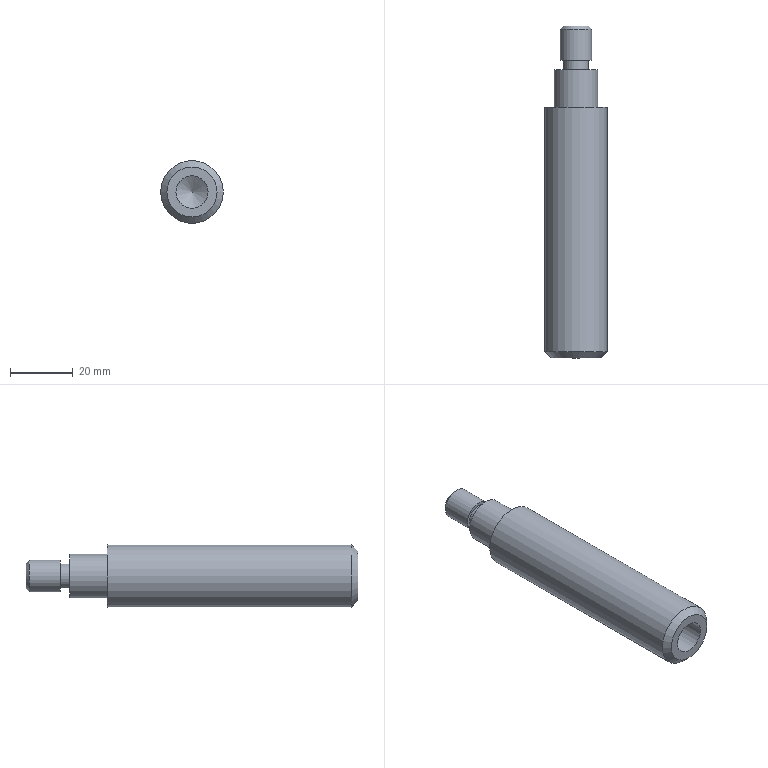Component | NX | PISTON_ROD | 1 solid | 13 faces | box 20 x 106 x 20 mm | volume 25777 mm3 | plane 5 | cylinder 5 | cone 3 | commonest cylinder face diameters 10 x1 8 x1 14 x1 20 x1 10.3 x1
STEP:
#1=CARTESIAN_POINT('',(0.,0.,0.));
#2=DIRECTION('',(0.,0.,1.));
#3=DIRECTION('',(1.,0.,0.));
#4=AXIS2_PLACEMENT_3D('',#1,#2,#3);
#5=CARTESIAN_POINT('',(4.,56.,43.));
#6=VERTEX_POINT('',#5);
#7=CARTESIAN_POINT('',(0.,56.,43.));
#8=DIRECTION('',(0.,-1.,0.));
#9=DIRECTION('',(1.,0.,0.));
#10=AXIS2_PLACEMENT_3D('',#7,#8,#9);
#11=CIRCLE('',#10,4.);
#12=CARTESIAN_POINT('',(0.,56.,43.));
#13=DIRECTION('',(0.,-1.,0.));
#14=DIRECTION('',(1.,0.,0.));
#15=AXIS2_PLACEMENT_3D('',#12,#13,#14);
#16=PLANE('',#15);
#17=CARTESIAN_POINT('',(0.,0.));
#18=DIRECTION('',(1.,0.));
#19=AXIS2_PLACEMENT_2D('',#17,#18);
#20=CIRCLE('',#19,4.);
#21=(GEOMETRIC_REPRESENTATION_CONTEXT(2)PARAMETRIC_REPRESENTATION_CONTEXT()REPRESENTATION_CONTEXT('',''));
#22=DEFINITIONAL_REPRESENTATION('',(#20),#21);
#23=PCURVE('',#16,#22);
#24=CARTESIAN_POINT('',(0.,56.,43.));
#25=DIRECTION('',(0.,-1.,0.));
#26=DIRECTION('',(1.,0.,0.));
#27=AXIS2_PLACEMENT_3D('',#24,#25,#26);
#28=CYLINDRICAL_SURFACE('',#27,4.);
#29=CARTESIAN_POINT('',(0.,0.));
#30=DIRECTION('',(1.,0.));
#31=VECTOR('',#30,1.);
#32=LINE('',#29,#31);
#33=(GEOMETRIC_REPRESENTATION_CONTEXT(2)PARAMETRIC_REPRESENTATION_CONTEXT()REPRESENTATION_CONTEXT('',''));
#34=DEFINITIONAL_REPRESENTATION('',(#32),#33);
#35=PCURVE('',#28,#34);
#36=SURFACE_CURVE('',#11,(#23,#35),.PCURVE_S1.);
#37=EDGE_CURVE('',#6,#6,#36,.T.);
#38=ORIENTED_EDGE('',*,*,#37,.F.);
#39=EDGE_LOOP('',(#38));
#40=FACE_BOUND('',#39,.T.);
#41=CARTESIAN_POINT('',(5.,56.,43.));
#42=VERTEX_POINT('',#41);
#43=CARTESIAN_POINT('',(0.,56.,43.));
#44=DIRECTION('',(0.,1.,0.));
#45=DIRECTION('',(1.,0.,0.));
#46=AXIS2_PLACEMENT_3D('',#43,#44,#45);
#47=CIRCLE('',#46,5.);
#48=CARTESIAN_POINT('',(5.,0.));
#49=CARTESIAN_POINT('',(5.,-8.66));
#50=CARTESIAN_POINT('',(-2.5,-4.33));
#51=CARTESIAN_POINT('',(-10.,-0.));
#52=CARTESIAN_POINT('',(-2.5,4.33));
#53=CARTESIAN_POINT('',(5.,8.66));
#54=CARTESIAN_POINT('',(5.,0.));
#55=(BOUNDED_CURVE()B_SPLINE_CURVE(2,(#48,#49,#50,#51,#52,#53,#54),.UNSPECIFIED.,.T.,.F.)B_SPLINE_CURVE_WITH_KNOTS((1,2,2,2,2,1),(-2.094,0.,2.094,4.189,6.283,8.378),.UNSPECIFIED.)CURVE()GEOMETRIC_REPRESENTATION_ITEM()RATIONAL_B_SPLINE_CURVE((1.,0.5,1.,0.5,1.,0.5,1.))REPRESENTATION_ITEM(''));
#56=(GEOMETRIC_REPRESENTATION_CONTEXT(2)PARAMETRIC_REPRESENTATION_CONTEXT()REPRESENTATION_CONTEXT('',''));
#57=DEFINITIONAL_REPRESENTATION('',(#55),#56);
#58=PCURVE('',#16,#57);
#59=CARTESIAN_POINT('',(0.,67.,43.));
#60=DIRECTION('',(0.,-1.,0.));
#61=DIRECTION('',(1.,0.,0.));
#62=AXIS2_PLACEMENT_3D('',#59,#60,#61);
#63=CYLINDRICAL_SURFACE('',#62,5.);
#64=CARTESIAN_POINT('',(6.283,11.));
#65=DIRECTION('',(-1.,0.));
#66=VECTOR('',#65,1.);
#67=LINE('',#64,#66);
#68=(GEOMETRIC_REPRESENTATION_CONTEXT(2)PARAMETRIC_REPRESENTATION_CONTEXT()REPRESENTATION_CONTEXT('',''));
#69=DEFINITIONAL_REPRESENTATION('',(#67),#68);
#70=PCURVE('',#63,#69);
#71=SURFACE_CURVE('',#47,(#58,#70),.PCURVE_S1.);
#72=EDGE_CURVE('',#42,#42,#71,.T.);
#73=ORIENTED_EDGE('',*,*,#72,.F.);
#74=EDGE_LOOP('',(#73));
#75=FACE_BOUND('',#74,.T.);
#76=ADVANCED_FACE('',(#40,#75),#16,.T.);
#77=CARTESIAN_POINT('',(-4.,67.,43.));
#78=VERTEX_POINT('',#77);
#79=CARTESIAN_POINT('',(0.,67.,43.));
#80=DIRECTION('',(0.,1.,0.));
#81=DIRECTION('',(-1.,0.,0.));
#82=AXIS2_PLACEMENT_3D('',#79,#80,#81);
#83=CIRCLE('',#82,4.);
#84=CARTESIAN_POINT('',(0.,67.,43.));
#85=DIRECTION('',(0.,1.,0.));
#86=DIRECTION('',(-1.,0.,0.));
#87=AXIS2_PLACEMENT_3D('',#84,#85,#86);
#88=PLANE('',#87);
#89=CARTESIAN_POINT('',(0.,0.));
#90=DIRECTION('',(1.,0.));
#91=AXIS2_PLACEMENT_2D('',#89,#90);
#92=CIRCLE('',#91,4.);
#93=(GEOMETRIC_REPRESENTATION_CONTEXT(2)PARAMETRIC_REPRESENTATION_CONTEXT()REPRESENTATION_CONTEXT('',''));
#94=DEFINITIONAL_REPRESENTATION('',(#92),#93);
#95=PCURVE('',#88,#94);
#96=CARTESIAN_POINT('',(0.,66.,43.));
#97=DIRECTION('',(0.,-1.,0.));
#98=DIRECTION('',(1.,0.,0.));
#99=AXIS2_PLACEMENT_3D('',#96,#97,#98);
#100=CONICAL_SURFACE('',#99,5.,0.7854);
#101=CARTESIAN_POINT('',(9.425,-1.));
#102=DIRECTION('',(-1.,0.));
#103=VECTOR('',#102,1.);
#104=LINE('',#101,#103);
#105=(GEOMETRIC_REPRESENTATION_CONTEXT(2)PARAMETRIC_REPRESENTATION_CONTEXT()REPRESENTATION_CONTEXT('',''));
#106=DEFINITIONAL_REPRESENTATION('',(#104),#105);
#107=PCURVE('',#100,#106);
#108=SURFACE_CURVE('',#83,(#95,#107),.PCURVE_S1.);
#109=EDGE_CURVE('',#78,#78,#108,.T.);
#110=ORIENTED_EDGE('',*,*,#109,.T.);
#111=EDGE_LOOP('',(#110));
#112=FACE_BOUND('',#111,.T.);
#113=ADVANCED_FACE('',(#112),#88,.T.);
#114=CARTESIAN_POINT('',(-5.,66.,43.));
#115=VERTEX_POINT('',#114);
#116=CARTESIAN_POINT('',(5.,66.,43.));
#117=VERTEX_POINT('',#116);
#118=CARTESIAN_POINT('',(0.,66.,43.));
#119=DIRECTION('',(0.,-1.,0.));
#120=DIRECTION('',(-1.,0.,0.));
#121=AXIS2_PLACEMENT_3D('',#118,#119,#120);
#122=CIRCLE('',#121,5.);
#123=CARTESIAN_POINT('',(3.142,1.));
#124=DIRECTION('',(1.,0.));
#125=VECTOR('',#124,1.);
#126=LINE('',#123,#125);
#127=(GEOMETRIC_REPRESENTATION_CONTEXT(2)PARAMETRIC_REPRESENTATION_CONTEXT()REPRESENTATION_CONTEXT('',''));
#128=DEFINITIONAL_REPRESENTATION('',(#126),#127);
#129=PCURVE('',#63,#128);
#130=CARTESIAN_POINT('',(3.142,0.));
#131=DIRECTION('',(1.,0.));
#132=VECTOR('',#131,1.);
#133=LINE('',#130,#132);
#134=(GEOMETRIC_REPRESENTATION_CONTEXT(2)PARAMETRIC_REPRESENTATION_CONTEXT()REPRESENTATION_CONTEXT('',''));
#135=DEFINITIONAL_REPRESENTATION('',(#133),#134);
#136=PCURVE('',#100,#135);
#137=SURFACE_CURVE('',#122,(#129,#136),.PCURVE_S1.);
#138=EDGE_CURVE('',#115,#117,#137,.T.);
#139=ORIENTED_EDGE('',*,*,#138,.T.);
#140=CARTESIAN_POINT('',(5.,66.,43.));
#141=CARTESIAN_POINT('',(5.,56.,43.));
#142=B_SPLINE_CURVE_WITH_KNOTS('',1,(#140,#141),.UNSPECIFIED.,.F.,.F.,(2,2),(1.,11.),.PIECEWISE_BEZIER_KNOTS.);
#143=CARTESIAN_POINT('',(6.283,0.));
#144=DIRECTION('',(0.,1.));
#145=VECTOR('',#144,1.);
#146=LINE('',#143,#145);
#147=(GEOMETRIC_REPRESENTATION_CONTEXT(2)PARAMETRIC_REPRESENTATION_CONTEXT()REPRESENTATION_CONTEXT('',''));
#148=DEFINITIONAL_REPRESENTATION('',(#146),#147);
#149=PCURVE('',#63,#148);
#150=CARTESIAN_POINT('',(0.,0.));
#151=DIRECTION('',(0.,1.));
#152=VECTOR('',#151,1.);
#153=LINE('',#150,#152);
#154=(GEOMETRIC_REPRESENTATION_CONTEXT(2)PARAMETRIC_REPRESENTATION_CONTEXT()REPRESENTATION_CONTEXT('',''));
#155=DEFINITIONAL_REPRESENTATION('',(#153),#154);
#156=PCURVE('',#63,#155);
#157=SEAM_CURVE('',#142,(#149,#156),.PCURVE_S1.);
#158=EDGE_CURVE('',#117,#42,#157,.T.);
#159=ORIENTED_EDGE('',*,*,#158,.T.);
#160=ORIENTED_EDGE('',*,*,#72,.T.);
#161=ORIENTED_EDGE('',*,*,#158,.F.);
#162=CARTESIAN_POINT('',(0.,66.,43.));
#163=DIRECTION('',(0.,-1.,0.));
#164=DIRECTION('',(-1.,0.,0.));
#165=AXIS2_PLACEMENT_3D('',#162,#163,#164);
#166=CIRCLE('',#165,5.);
#167=CARTESIAN_POINT('',(-3.142,1.));
#168=DIRECTION('',(1.,0.));
#169=VECTOR('',#168,1.);
#170=LINE('',#167,#169);
#171=(GEOMETRIC_REPRESENTATION_CONTEXT(2)PARAMETRIC_REPRESENTATION_CONTEXT()REPRESENTATION_CONTEXT('',''));
#172=DEFINITIONAL_REPRESENTATION('',(#170),#171);
#173=PCURVE('',#63,#172);
#174=CARTESIAN_POINT('',(3.142,0.));
#175=DIRECTION('',(1.,0.));
#176=VECTOR('',#175,1.);
#177=LINE('',#174,#176);
#178=(GEOMETRIC_REPRESENTATION_CONTEXT(2)PARAMETRIC_REPRESENTATION_CONTEXT()REPRESENTATION_CONTEXT('',''));
#179=DEFINITIONAL_REPRESENTATION('',(#177),#178);
#180=PCURVE('',#100,#179);
#181=SURFACE_CURVE('',#166,(#173,#180),.PCURVE_S1.);
#182=EDGE_CURVE('',#117,#115,#181,.T.);
#183=ORIENTED_EDGE('',*,*,#182,.T.);
#184=EDGE_LOOP('',(#139,#159,#160,#161,#183));
#185=FACE_BOUND('',#184,.T.);
#186=ADVANCED_FACE('',(#185),#63,.T.);
#187=CARTESIAN_POINT('',(4.,53.,43.));
#188=VERTEX_POINT('',#187);
#189=CARTESIAN_POINT('',(-4.,53.,43.));
#190=VERTEX_POINT('',#189);
#191=CARTESIAN_POINT('',(0.,53.,43.));
#192=DIRECTION('',(0.,-1.,0.));
#193=DIRECTION('',(-1.,0.,0.));
#194=AXIS2_PLACEMENT_3D('',#191,#192,#193);
#195=CIRCLE('',#194,4.);
#196=CARTESIAN_POINT('',(-3.142,3.));
#197=DIRECTION('',(1.,0.));
#198=VECTOR('',#197,1.);
#199=LINE('',#196,#198);
#200=(GEOMETRIC_REPRESENTATION_CONTEXT(2)PARAMETRIC_REPRESENTATION_CONTEXT()REPRESENTATION_CONTEXT('',''));
#201=DEFINITIONAL_REPRESENTATION('',(#199),#200);
#202=PCURVE('',#28,#201);
#203=CARTESIAN_POINT('',(0.,53.,43.));
#204=DIRECTION('',(0.,1.,0.));
#205=DIRECTION('',(-1.,0.,0.));
#206=AXIS2_PLACEMENT_3D('',#203,#204,#205);
#207=PLANE('',#206);
#208=CARTESIAN_POINT('',(4.,0.));
#209=CARTESIAN_POINT('',(4.,-6.928));
#210=CARTESIAN_POINT('',(-2.,-3.464));
#211=CARTESIAN_POINT('',(-8.,-0.));
#212=CARTESIAN_POINT('',(-2.,3.464));
#213=CARTESIAN_POINT('',(4.,6.928));
#214=CARTESIAN_POINT('',(4.,0.));
#215=(BOUNDED_CURVE()B_SPLINE_CURVE(2,(#208,#209,#210,#211,#212,#213,#214),.UNSPECIFIED.,.T.,.F.)B_SPLINE_CURVE_WITH_KNOTS((1,2,2,2,2,1),(-2.094,0.,2.094,4.189,6.283,8.378),.UNSPECIFIED.)CURVE()GEOMETRIC_REPRESENTATION_ITEM()RATIONAL_B_SPLINE_CURVE((1.,0.5,1.,0.5,1.,0.5,1.))REPRESENTATION_ITEM(''));
#216=(GEOMETRIC_REPRESENTATION_CONTEXT(2)PARAMETRIC_REPRESENTATION_CONTEXT()REPRESENTATION_CONTEXT('',''));
#217=DEFINITIONAL_REPRESENTATION('',(#215),#216);
#218=PCURVE('',#207,#217);
#219=SURFACE_CURVE('',#195,(#202,#218),.PCURVE_S1.);
#220=EDGE_CURVE('',#188,#190,#219,.T.);
#221=ORIENTED_EDGE('',*,*,#220,.F.);
#222=CARTESIAN_POINT('',(4.,56.,43.));
#223=CARTESIAN_POINT('',(4.,53.,43.));
#224=B_SPLINE_CURVE_WITH_KNOTS('',1,(#222,#223),.UNSPECIFIED.,.F.,.F.,(2,2),(0.,3.),.PIECEWISE_BEZIER_KNOTS.);
#225=CARTESIAN_POINT('',(0.,0.));
#226=DIRECTION('',(0.,1.));
#227=VECTOR('',#226,1.);
#228=LINE('',#225,#227);
#229=(GEOMETRIC_REPRESENTATION_CONTEXT(2)PARAMETRIC_REPRESENTATION_CONTEXT()REPRESENTATION_CONTEXT('',''));
#230=DEFINITIONAL_REPRESENTATION('',(#228),#229);
#231=PCURVE('',#28,#230);
#232=CARTESIAN_POINT('',(6.283,0.));
#233=DIRECTION('',(0.,1.));
#234=VECTOR('',#233,1.);
#235=LINE('',#232,#234);
#236=(GEOMETRIC_REPRESENTATION_CONTEXT(2)PARAMETRIC_REPRESENTATION_CONTEXT()REPRESENTATION_CONTEXT('',''));
#237=DEFINITIONAL_REPRESENTATION('',(#235),#236);
#238=PCURVE('',#28,#237);
#239=SEAM_CURVE('',#224,(#231,#238),.PCURVE_S1.);
#240=EDGE_CURVE('',#6,#188,#239,.T.);
#241=ORIENTED_EDGE('',*,*,#240,.F.);
#242=ORIENTED_EDGE('',*,*,#37,.T.);
#243=ORIENTED_EDGE('',*,*,#240,.T.);
#244=CARTESIAN_POINT('',(0.,53.,43.));
#245=DIRECTION('',(0.,-1.,0.));
#246=DIRECTION('',(-1.,0.,0.));
#247=AXIS2_PLACEMENT_3D('',#244,#245,#246);
#248=CIRCLE('',#247,4.);
#249=CARTESIAN_POINT('',(3.142,3.));
#250=DIRECTION('',(1.,0.));
#251=VECTOR('',#250,1.);
#252=LINE('',#249,#251);
#253=(GEOMETRIC_REPRESENTATION_CONTEXT(2)PARAMETRIC_REPRESENTATION_CONTEXT()REPRESENTATION_CONTEXT('',''));
#254=DEFINITIONAL_REPRESENTATION('',(#252),#253);
#255=PCURVE('',#28,#254);
#256=CARTESIAN_POINT('',(4.,0.));
#257=CARTESIAN_POINT('',(4.,-6.928));
#258=CARTESIAN_POINT('',(-2.,-3.464));
#259=CARTESIAN_POINT('',(-8.,-0.));
#260=CARTESIAN_POINT('',(-2.,3.464));
#261=CARTESIAN_POINT('',(4.,6.928));
#262=CARTESIAN_POINT('',(4.,0.));
#263=(BOUNDED_CURVE()B_SPLINE_CURVE(2,(#256,#257,#258,#259,#260,#261,#262),.UNSPECIFIED.,.T.,.F.)B_SPLINE_CURVE_WITH_KNOTS((1,2,2,2,2,1),(-2.094,0.,2.094,4.189,6.283,8.378),.UNSPECIFIED.)CURVE()GEOMETRIC_REPRESENTATION_ITEM()RATIONAL_B_SPLINE_CURVE((1.,0.5,1.,0.5,1.,0.5,1.))REPRESENTATION_ITEM(''));
#264=(GEOMETRIC_REPRESENTATION_CONTEXT(2)PARAMETRIC_REPRESENTATION_CONTEXT()REPRESENTATION_CONTEXT('',''));
#265=DEFINITIONAL_REPRESENTATION('',(#263),#264);
#266=PCURVE('',#207,#265);
#267=SURFACE_CURVE('',#248,(#255,#266),.PCURVE_S1.);
#268=EDGE_CURVE('',#190,#188,#267,.T.);
#269=ORIENTED_EDGE('',*,*,#268,.F.);
#270=EDGE_LOOP('',(#221,#241,#242,#243,#269));
#271=FACE_BOUND('',#270,.T.);
#272=ADVANCED_FACE('',(#271),#28,.T.);
#273=ORIENTED_EDGE('',*,*,#268,.T.);
#274=ORIENTED_EDGE('',*,*,#220,.T.);
#275=EDGE_LOOP('',(#273,#274));
#276=FACE_BOUND('',#275,.T.);
#277=CARTESIAN_POINT('',(7.,53.,43.));
#278=VERTEX_POINT('',#277);
#279=CARTESIAN_POINT('',(0.,53.,43.));
#280=DIRECTION('',(0.,-1.,0.));
#281=DIRECTION('',(1.,0.,0.));
#282=AXIS2_PLACEMENT_3D('',#279,#280,#281);
#283=CIRCLE('',#282,7.);
#284=CARTESIAN_POINT('',(-7.,0.));
#285=CARTESIAN_POINT('',(-7.,12.124));
#286=CARTESIAN_POINT('',(3.5,6.062));
#287=CARTESIAN_POINT('',(14.,0.));
#288=CARTESIAN_POINT('',(3.5,-6.062));
#289=CARTESIAN_POINT('',(-7.,-12.124));
#290=CARTESIAN_POINT('',(-7.,0.));
#291=(BOUNDED_CURVE()B_SPLINE_CURVE(2,(#284,#285,#286,#287,#288,#289,#290),.UNSPECIFIED.,.T.,.F.)B_SPLINE_CURVE_WITH_KNOTS((1,2,2,2,2,1),(-2.094,0.,2.094,4.189,6.283,8.378),.UNSPECIFIED.)CURVE()GEOMETRIC_REPRESENTATION_ITEM()RATIONAL_B_SPLINE_CURVE((1.,0.5,1.,0.5,1.,0.5,1.))REPRESENTATION_ITEM(''));
#292=(GEOMETRIC_REPRESENTATION_CONTEXT(2)PARAMETRIC_REPRESENTATION_CONTEXT()REPRESENTATION_CONTEXT('',''));
#293=DEFINITIONAL_REPRESENTATION('',(#291),#292);
#294=PCURVE('',#207,#293);
#295=CARTESIAN_POINT('',(0.,53.,43.));
#296=DIRECTION('',(0.,-1.,0.));
#297=DIRECTION('',(1.,0.,0.));
#298=AXIS2_PLACEMENT_3D('',#295,#296,#297);
#299=CYLINDRICAL_SURFACE('',#298,7.);
#300=CARTESIAN_POINT('',(0.,0.));
#301=DIRECTION('',(1.,0.));
#302=VECTOR('',#301,1.);
#303=LINE('',#300,#302);
#304=(GEOMETRIC_REPRESENTATION_CONTEXT(2)PARAMETRIC_REPRESENTATION_CONTEXT()REPRESENTATION_CONTEXT('',''));
#305=DEFINITIONAL_REPRESENTATION('',(#303),#304);
#306=PCURVE('',#299,#305);
#307=SURFACE_CURVE('',#283,(#294,#306),.PCURVE_S1.);
#308=EDGE_CURVE('',#278,#278,#307,.T.);
#309=ORIENTED_EDGE('',*,*,#308,.F.);
#310=EDGE_LOOP('',(#309));
#311=FACE_BOUND('',#310,.T.);
#312=ADVANCED_FACE('',(#276,#311),#207,.T.);
#313=CARTESIAN_POINT('',(7.,41.,43.));
#314=VERTEX_POINT('',#313);
#315=CARTESIAN_POINT('',(-7.,41.,43.));
#316=VERTEX_POINT('',#315);
#317=CARTESIAN_POINT('',(0.,41.,43.));
#318=DIRECTION('',(0.,-1.,0.));
#319=DIRECTION('',(-1.,0.,0.));
#320=AXIS2_PLACEMENT_3D('',#317,#318,#319);
#321=CIRCLE('',#320,7.);
#322=CARTESIAN_POINT('',(-3.142,12.));
#323=DIRECTION('',(1.,0.));
#324=VECTOR('',#323,1.);
#325=LINE('',#322,#324);
#326=(GEOMETRIC_REPRESENTATION_CONTEXT(2)PARAMETRIC_REPRESENTATION_CONTEXT()REPRESENTATION_CONTEXT('',''));
#327=DEFINITIONAL_REPRESENTATION('',(#325),#326);
#328=PCURVE('',#299,#327);
#329=CARTESIAN_POINT('',(0.,41.,43.));
#330=DIRECTION('',(0.,1.,0.));
#331=DIRECTION('',(-1.,0.,0.));
#332=AXIS2_PLACEMENT_3D('',#329,#330,#331);
#333=PLANE('',#332);
#334=CARTESIAN_POINT('',(7.,0.));
#335=CARTESIAN_POINT('',(7.,-12.124));
#336=CARTESIAN_POINT('',(-3.5,-6.062));
#337=CARTESIAN_POINT('',(-14.,-0.));
#338=CARTESIAN_POINT('',(-3.5,6.062));
#339=CARTESIAN_POINT('',(7.,12.124));
#340=CARTESIAN_POINT('',(7.,0.));
#341=(BOUNDED_CURVE()B_SPLINE_CURVE(2,(#334,#335,#336,#337,#338,#339,#340),.UNSPECIFIED.,.T.,.F.)B_SPLINE_CURVE_WITH_KNOTS((1,2,2,2,2,1),(-2.094,0.,2.094,4.189,6.283,8.378),.UNSPECIFIED.)CURVE()GEOMETRIC_REPRESENTATION_ITEM()RATIONAL_B_SPLINE_CURVE((1.,0.5,1.,0.5,1.,0.5,1.))REPRESENTATION_ITEM(''));
#342=(GEOMETRIC_REPRESENTATION_CONTEXT(2)PARAMETRIC_REPRESENTATION_CONTEXT()REPRESENTATION_CONTEXT('',''));
#343=DEFINITIONAL_REPRESENTATION('',(#341),#342);
#344=PCURVE('',#333,#343);
#345=SURFACE_CURVE('',#321,(#328,#344),.PCURVE_S1.);
#346=EDGE_CURVE('',#314,#316,#345,.T.);
#347=ORIENTED_EDGE('',*,*,#346,.F.);
#348=CARTESIAN_POINT('',(7.,53.,43.));
#349=CARTESIAN_POINT('',(7.,41.,43.));
#350=B_SPLINE_CURVE_WITH_KNOTS('',1,(#348,#349),.UNSPECIFIED.,.F.,.F.,(2,2),(0.,12.),.PIECEWISE_BEZIER_KNOTS.);
#351=CARTESIAN_POINT('',(0.,0.));
#352=DIRECTION('',(0.,1.));
#353=VECTOR('',#352,1.);
#354=LINE('',#351,#353);
#355=(GEOMETRIC_REPRESENTATION_CONTEXT(2)PARAMETRIC_REPRESENTATION_CONTEXT()REPRESENTATION_CONTEXT('',''));
#356=DEFINITIONAL_REPRESENTATION('',(#354),#355);
#357=PCURVE('',#299,#356);
#358=CARTESIAN_POINT('',(6.283,0.));
#359=DIRECTION('',(0.,1.));
#360=VECTOR('',#359,1.);
#361=LINE('',#358,#360);
#362=(GEOMETRIC_REPRESENTATION_CONTEXT(2)PARAMETRIC_REPRESENTATION_CONTEXT()REPRESENTATION_CONTEXT('',''));
#363=DEFINITIONAL_REPRESENTATION('',(#361),#362);
#364=PCURVE('',#299,#363);
#365=SEAM_CURVE('',#350,(#357,#364),.PCURVE_S1.);
#366=EDGE_CURVE('',#278,#314,#365,.T.);
#367=ORIENTED_EDGE('',*,*,#366,.F.);
#368=ORIENTED_EDGE('',*,*,#308,.T.);
#369=ORIENTED_EDGE('',*,*,#366,.T.);
#370=CARTESIAN_POINT('',(0.,41.,43.));
#371=DIRECTION('',(0.,-1.,0.));
#372=DIRECTION('',(-1.,0.,0.));
#373=AXIS2_PLACEMENT_3D('',#370,#371,#372);
#374=CIRCLE('',#373,7.);
#375=CARTESIAN_POINT('',(3.142,12.));
#376=DIRECTION('',(1.,0.));
#377=VECTOR('',#376,1.);
#378=LINE('',#375,#377);
#379=(GEOMETRIC_REPRESENTATION_CONTEXT(2)PARAMETRIC_REPRESENTATION_CONTEXT()REPRESENTATION_CONTEXT('',''));
#380=DEFINITIONAL_REPRESENTATION('',(#378),#379);
#381=PCURVE('',#299,#380);
#382=CARTESIAN_POINT('',(7.,0.));
#383=CARTESIAN_POINT('',(7.,-12.124));
#384=CARTESIAN_POINT('',(-3.5,-6.062));
#385=CARTESIAN_POINT('',(-14.,-0.));
#386=CARTESIAN_POINT('',(-3.5,6.062));
#387=CARTESIAN_POINT('',(7.,12.124));
#388=CARTESIAN_POINT('',(7.,0.));
#389=(BOUNDED_CURVE()B_SPLINE_CURVE(2,(#382,#383,#384,#385,#386,#387,#388),.UNSPECIFIED.,.T.,.F.)B_SPLINE_CURVE_WITH_KNOTS((1,2,2,2,2,1),(-2.094,0.,2.094,4.189,6.283,8.378),.UNSPECIFIED.)CURVE()GEOMETRIC_REPRESENTATION_ITEM()RATIONAL_B_SPLINE_CURVE((1.,0.5,1.,0.5,1.,0.5,1.))REPRESENTATION_ITEM(''));
#390=(GEOMETRIC_REPRESENTATION_CONTEXT(2)PARAMETRIC_REPRESENTATION_CONTEXT()REPRESENTATION_CONTEXT('',''));
#391=DEFINITIONAL_REPRESENTATION('',(#389),#390);
#392=PCURVE('',#333,#391);
#393=SURFACE_CURVE('',#374,(#381,#392),.PCURVE_S1.);
#394=EDGE_CURVE('',#316,#314,#393,.T.);
#395=ORIENTED_EDGE('',*,*,#394,.F.);
#396=EDGE_LOOP('',(#347,#367,#368,#369,#395));
#397=FACE_BOUND('',#396,.T.);
#398=ADVANCED_FACE('',(#397),#299,.T.);
#399=CARTESIAN_POINT('',(-5.15,-39.,43.));
#400=VERTEX_POINT('',#399);
#401=CARTESIAN_POINT('',(0.,-39.,43.));
#402=DIRECTION('',(0.,1.,0.));
#403=DIRECTION('',(-1.,0.,0.));
#404=AXIS2_PLACEMENT_3D('',#401,#402,#403);
#405=CIRCLE('',#404,5.15);
#406=CARTESIAN_POINT('',(0.,-39.,43.));
#407=DIRECTION('',(0.,-1.,0.));
#408=DIRECTION('',(1.,0.,0.));
#409=AXIS2_PLACEMENT_3D('',#406,#407,#408);
#410=PLANE('',#409);
#411=CARTESIAN_POINT('',(-5.15,0.));
#412=CARTESIAN_POINT('',(-5.15,8.92));
#413=CARTESIAN_POINT('',(2.575,4.46));
#414=CARTESIAN_POINT('',(10.3,0.));
#415=CARTESIAN_POINT('',(2.575,-4.46));
#416=CARTESIAN_POINT('',(-5.15,-8.92));
#417=CARTESIAN_POINT('',(-5.15,0.));
#418=(BOUNDED_CURVE()B_SPLINE_CURVE(2,(#411,#412,#413,#414,#415,#416,#417),.UNSPECIFIED.,.T.,.F.)B_SPLINE_CURVE_WITH_KNOTS((1,2,2,2,2,1),(-2.094,0.,2.094,4.189,6.283,8.378),.UNSPECIFIED.)CURVE()GEOMETRIC_REPRESENTATION_ITEM()RATIONAL_B_SPLINE_CURVE((1.,0.5,1.,0.5,1.,0.5,1.))REPRESENTATION_ITEM(''));
#419=(GEOMETRIC_REPRESENTATION_CONTEXT(2)PARAMETRIC_REPRESENTATION_CONTEXT()REPRESENTATION_CONTEXT('',''));
#420=DEFINITIONAL_REPRESENTATION('',(#418),#419);
#421=PCURVE('',#410,#420);
#422=CARTESIAN_POINT('',(0.,-39.,43.));
#423=DIRECTION('',(0.,1.,0.));
#424=DIRECTION('',(-1.,0.,0.));
#425=AXIS2_PLACEMENT_3D('',#422,#423,#424);
#426=CYLINDRICAL_SURFACE('',#425,5.15);
#427=CARTESIAN_POINT('',(0.,0.));
#428=DIRECTION('',(1.,0.));
#429=VECTOR('',#428,1.);
#430=LINE('',#427,#429);
#431=(GEOMETRIC_REPRESENTATION_CONTEXT(2)PARAMETRIC_REPRESENTATION_CONTEXT()REPRESENTATION_CONTEXT('',''));
#432=DEFINITIONAL_REPRESENTATION('',(#430),#431);
#433=PCURVE('',#426,#432);
#434=SURFACE_CURVE('',#405,(#421,#433),.PCURVE_S1.);
#435=EDGE_CURVE('',#400,#400,#434,.T.);
#436=ORIENTED_EDGE('',*,*,#435,.T.);
#437=EDGE_LOOP('',(#436));
#438=FACE_BOUND('',#437,.T.);
#439=CARTESIAN_POINT('',(8.,-39.,43.));
#440=VERTEX_POINT('',#439);
#441=CARTESIAN_POINT('',(0.,-39.,43.));
#442=DIRECTION('',(0.,-1.,0.));
#443=DIRECTION('',(1.,0.,0.));
#444=AXIS2_PLACEMENT_3D('',#441,#442,#443);
#445=CIRCLE('',#444,8.);
#446=CARTESIAN_POINT('',(0.,0.));
#447=DIRECTION('',(1.,0.));
#448=AXIS2_PLACEMENT_2D('',#446,#447);
#449=CIRCLE('',#448,8.);
#450=(GEOMETRIC_REPRESENTATION_CONTEXT(2)PARAMETRIC_REPRESENTATION_CONTEXT()REPRESENTATION_CONTEXT('',''));
#451=DEFINITIONAL_REPRESENTATION('',(#449),#450);
#452=PCURVE('',#410,#451);
#453=CARTESIAN_POINT('',(0.,-37.,43.));
#454=DIRECTION('',(0.,1.,0.));
#455=DIRECTION('',(-1.,0.,0.));
#456=AXIS2_PLACEMENT_3D('',#453,#454,#455);
#457=CONICAL_SURFACE('',#456,10.,0.7854);
#458=CARTESIAN_POINT('',(9.425,-2.));
#459=DIRECTION('',(-1.,0.));
#460=VECTOR('',#459,1.);
#461=LINE('',#458,#460);
#462=(GEOMETRIC_REPRESENTATION_CONTEXT(2)PARAMETRIC_REPRESENTATION_CONTEXT()REPRESENTATION_CONTEXT('',''));
#463=DEFINITIONAL_REPRESENTATION('',(#461),#462);
#464=PCURVE('',#457,#463);
#465=SURFACE_CURVE('',#445,(#452,#464),.PCURVE_S1.);
#466=EDGE_CURVE('',#440,#440,#465,.T.);
#467=ORIENTED_EDGE('',*,*,#466,.T.);
#468=EDGE_LOOP('',(#467));
#469=FACE_BOUND('',#468,.T.);
#470=ADVANCED_FACE('',(#438,#469),#410,.T.);
#471=ORIENTED_EDGE('',*,*,#394,.T.);
#472=ORIENTED_EDGE('',*,*,#346,.T.);
#473=EDGE_LOOP('',(#471,#472));
#474=FACE_BOUND('',#473,.T.);
#475=CARTESIAN_POINT('',(10.,41.,43.));
#476=VERTEX_POINT('',#475);
#477=CARTESIAN_POINT('',(0.,41.,43.));
#478=DIRECTION('',(0.,-1.,0.));
#479=DIRECTION('',(1.,0.,0.));
#480=AXIS2_PLACEMENT_3D('',#477,#478,#479);
#481=CIRCLE('',#480,10.);
#482=CARTESIAN_POINT('',(-10.,0.));
#483=CARTESIAN_POINT('',(-10.,17.321));
#484=CARTESIAN_POINT('',(5.,8.66));
#485=CARTESIAN_POINT('',(20.,0.));
#486=CARTESIAN_POINT('',(5.,-8.66));
#487=CARTESIAN_POINT('',(-10.,-17.321));
#488=CARTESIAN_POINT('',(-10.,0.));
#489=(BOUNDED_CURVE()B_SPLINE_CURVE(2,(#482,#483,#484,#485,#486,#487,#488),.UNSPECIFIED.,.T.,.F.)B_SPLINE_CURVE_WITH_KNOTS((1,2,2,2,2,1),(-2.094,0.,2.094,4.189,6.283,8.378),.UNSPECIFIED.)CURVE()GEOMETRIC_REPRESENTATION_ITEM()RATIONAL_B_SPLINE_CURVE((1.,0.5,1.,0.5,1.,0.5,1.))REPRESENTATION_ITEM(''));
#490=(GEOMETRIC_REPRESENTATION_CONTEXT(2)PARAMETRIC_REPRESENTATION_CONTEXT()REPRESENTATION_CONTEXT('',''));
#491=DEFINITIONAL_REPRESENTATION('',(#489),#490);
#492=PCURVE('',#333,#491);
#493=CARTESIAN_POINT('',(0.,41.,43.));
#494=DIRECTION('',(0.,-1.,0.));
#495=DIRECTION('',(1.,0.,0.));
#496=AXIS2_PLACEMENT_3D('',#493,#494,#495);
#497=CYLINDRICAL_SURFACE('',#496,10.);
#498=CARTESIAN_POINT('',(0.,0.));
#499=DIRECTION('',(1.,0.));
#500=VECTOR('',#499,1.);
#501=LINE('',#498,#500);
#502=(GEOMETRIC_REPRESENTATION_CONTEXT(2)PARAMETRIC_REPRESENTATION_CONTEXT()REPRESENTATION_CONTEXT('',''));
#503=DEFINITIONAL_REPRESENTATION('',(#501),#502);
#504=PCURVE('',#497,#503);
#505=SURFACE_CURVE('',#481,(#492,#504),.PCURVE_S1.);
#506=EDGE_CURVE('',#476,#476,#505,.T.);
#507=ORIENTED_EDGE('',*,*,#506,.F.);
#508=EDGE_LOOP('',(#507));
#509=FACE_BOUND('',#508,.T.);
#510=ADVANCED_FACE('',(#474,#509),#333,.T.);
#511=CARTESIAN_POINT('',(10.,-37.,43.));
#512=VERTEX_POINT('',#511);
#513=CARTESIAN_POINT('',(0.,-37.,43.));
#514=DIRECTION('',(0.,1.,0.));
#515=DIRECTION('',(1.,0.,0.));
#516=AXIS2_PLACEMENT_3D('',#513,#514,#515);
#517=CIRCLE('',#516,10.);
#518=CARTESIAN_POINT('',(6.283,78.));
#519=DIRECTION('',(-1.,0.));
#520=VECTOR('',#519,1.);
#521=LINE('',#518,#520);
#522=(GEOMETRIC_REPRESENTATION_CONTEXT(2)PARAMETRIC_REPRESENTATION_CONTEXT()REPRESENTATION_CONTEXT('',''));
#523=DEFINITIONAL_REPRESENTATION('',(#521),#522);
#524=PCURVE('',#497,#523);
#525=CARTESIAN_POINT('',(3.142,0.));
#526=DIRECTION('',(1.,0.));
#527=VECTOR('',#526,1.);
#528=LINE('',#525,#527);
#529=(GEOMETRIC_REPRESENTATION_CONTEXT(2)PARAMETRIC_REPRESENTATION_CONTEXT()REPRESENTATION_CONTEXT('',''));
#530=DEFINITIONAL_REPRESENTATION('',(#528),#529);
#531=PCURVE('',#457,#530);
#532=SURFACE_CURVE('',#517,(#524,#531),.PCURVE_S1.);
#533=EDGE_CURVE('',#512,#512,#532,.T.);
#534=ORIENTED_EDGE('',*,*,#533,.T.);
#535=CARTESIAN_POINT('',(10.,41.,43.));
#536=CARTESIAN_POINT('',(10.,-37.,43.));
#537=B_SPLINE_CURVE_WITH_KNOTS('',1,(#535,#536),.UNSPECIFIED.,.F.,.F.,(2,2),(0.,78.),.PIECEWISE_BEZIER_KNOTS.);
#538=CARTESIAN_POINT('',(0.,0.));
#539=DIRECTION('',(0.,1.));
#540=VECTOR('',#539,1.);
#541=LINE('',#538,#540);
#542=(GEOMETRIC_REPRESENTATION_CONTEXT(2)PARAMETRIC_REPRESENTATION_CONTEXT()REPRESENTATION_CONTEXT('',''));
#543=DEFINITIONAL_REPRESENTATION('',(#541),#542);
#544=PCURVE('',#497,#543);
#545=CARTESIAN_POINT('',(6.283,0.));
#546=DIRECTION('',(0.,1.));
#547=VECTOR('',#546,1.);
#548=LINE('',#545,#547);
#549=(GEOMETRIC_REPRESENTATION_CONTEXT(2)PARAMETRIC_REPRESENTATION_CONTEXT()REPRESENTATION_CONTEXT('',''));
#550=DEFINITIONAL_REPRESENTATION('',(#548),#549);
#551=PCURVE('',#497,#550);
#552=SEAM_CURVE('',#537,(#544,#551),.PCURVE_S1.);
#553=EDGE_CURVE('',#476,#512,#552,.T.);
#554=ORIENTED_EDGE('',*,*,#553,.F.);
#555=ORIENTED_EDGE('',*,*,#506,.T.);
#556=ORIENTED_EDGE('',*,*,#553,.T.);
#557=EDGE_LOOP('',(#534,#554,#555,#556));
#558=FACE_BOUND('',#557,.T.);
#559=ADVANCED_FACE('',(#558),#497,.T.);
#560=ORIENTED_EDGE('',*,*,#466,.F.);
#561=CARTESIAN_POINT('',(8.,-39.,43.));
#562=CARTESIAN_POINT('',(10.,-37.,43.));
#563=B_SPLINE_CURVE_WITH_KNOTS('',1,(#561,#562),.UNSPECIFIED.,.F.,.F.,(2,2),(-2.828,0.),.PIECEWISE_BEZIER_KNOTS.);
#564=CARTESIAN_POINT('',(9.425,0.));
#565=DIRECTION('',(0.,1.));
#566=VECTOR('',#565,1.);
#567=LINE('',#564,#566);
#568=(GEOMETRIC_REPRESENTATION_CONTEXT(2)PARAMETRIC_REPRESENTATION_CONTEXT()REPRESENTATION_CONTEXT('',''));
#569=DEFINITIONAL_REPRESENTATION('',(#567),#568);
#570=PCURVE('',#457,#569);
#571=CARTESIAN_POINT('',(3.142,0.));
#572=DIRECTION('',(0.,1.));
#573=VECTOR('',#572,1.);
#574=LINE('',#571,#573);
#575=(GEOMETRIC_REPRESENTATION_CONTEXT(2)PARAMETRIC_REPRESENTATION_CONTEXT()REPRESENTATION_CONTEXT('',''));
#576=DEFINITIONAL_REPRESENTATION('',(#574),#575);
#577=PCURVE('',#457,#576);
#578=SEAM_CURVE('',#563,(#570,#577),.PCURVE_S1.);
#579=EDGE_CURVE('',#440,#512,#578,.T.);
#580=ORIENTED_EDGE('',*,*,#579,.T.);
#581=ORIENTED_EDGE('',*,*,#533,.F.);
#582=ORIENTED_EDGE('',*,*,#579,.F.);
#583=EDGE_LOOP('',(#560,#580,#581,#582));
#584=FACE_BOUND('',#583,.T.);
#585=ADVANCED_FACE('',(#584),#457,.T.);
#586=CARTESIAN_POINT('',(5.15,-15.,43.));
#587=VERTEX_POINT('',#586);
#588=CARTESIAN_POINT('',(-5.15,-15.,43.));
#589=VERTEX_POINT('',#588);
#590=CARTESIAN_POINT('',(0.,-15.,43.));
#591=DIRECTION('',(0.,-1.,0.));
#592=DIRECTION('',(-1.,0.,0.));
#593=AXIS2_PLACEMENT_3D('',#590,#591,#592);
#594=CIRCLE('',#593,5.15);
#595=CARTESIAN_POINT('',(0.,-15.,43.));
#596=DIRECTION('',(0.,-1.,0.));
#597=DIRECTION('',(1.,0.,0.));
#598=AXIS2_PLACEMENT_3D('',#595,#596,#597);
#599=CONICAL_SURFACE('',#598,5.15,1.03);
#600=CARTESIAN_POINT('',(-3.142,0.));
#601=DIRECTION('',(1.,0.));
#602=VECTOR('',#601,1.);
#603=LINE('',#600,#602);
#604=(GEOMETRIC_REPRESENTATION_CONTEXT(2)PARAMETRIC_REPRESENTATION_CONTEXT()REPRESENTATION_CONTEXT('',''));
#605=DEFINITIONAL_REPRESENTATION('',(#603),#604);
#606=PCURVE('',#599,#605);
#607=CARTESIAN_POINT('',(6.283,24.));
#608=DIRECTION('',(-1.,0.));
#609=VECTOR('',#608,1.);
#610=LINE('',#607,#609);
#611=(GEOMETRIC_REPRESENTATION_CONTEXT(2)PARAMETRIC_REPRESENTATION_CONTEXT()REPRESENTATION_CONTEXT('',''));
#612=DEFINITIONAL_REPRESENTATION('',(#610),#611);
#613=PCURVE('',#426,#612);
#614=SURFACE_CURVE('',#594,(#606,#613),.PCURVE_S1.);
#615=EDGE_CURVE('',#587,#589,#614,.T.);
#616=ORIENTED_EDGE('',*,*,#615,.F.);
#617=CARTESIAN_POINT('',(0.,-11.906,43.));
#618=VERTEX_POINT('',#617);
#619=CARTESIAN_POINT('',(0.,-11.906,43.));
#620=CARTESIAN_POINT('',(5.15,-15.,43.));
#621=B_SPLINE_CURVE_WITH_KNOTS('',1,(#619,#620),.UNSPECIFIED.,.F.,.F.,(2,2),(-6.008,0.),.PIECEWISE_BEZIER_KNOTS.);
#622=CARTESIAN_POINT('',(0.,0.));
#623=DIRECTION('',(0.,1.));
#624=VECTOR('',#623,1.);
#625=LINE('',#622,#624);
#626=(GEOMETRIC_REPRESENTATION_CONTEXT(2)PARAMETRIC_REPRESENTATION_CONTEXT()REPRESENTATION_CONTEXT('',''));
#627=DEFINITIONAL_REPRESENTATION('',(#625),#626);
#628=PCURVE('',#599,#627);
#629=CARTESIAN_POINT('',(6.283,0.));
#630=DIRECTION('',(0.,1.));
#631=VECTOR('',#630,1.);
#632=LINE('',#629,#631);
#633=(GEOMETRIC_REPRESENTATION_CONTEXT(2)PARAMETRIC_REPRESENTATION_CONTEXT()REPRESENTATION_CONTEXT('',''));
#634=DEFINITIONAL_REPRESENTATION('',(#632),#633);
#635=PCURVE('',#599,#634);
#636=SEAM_CURVE('',#621,(#628,#635),.PCURVE_S1.);
#637=EDGE_CURVE('',#618,#587,#636,.T.);
#638=ORIENTED_EDGE('',*,*,#637,.F.);
#639=ORIENTED_EDGE('',*,*,#637,.T.);
#640=CARTESIAN_POINT('',(0.,-15.,43.));
#641=DIRECTION('',(0.,-1.,0.));
#642=DIRECTION('',(-1.,0.,0.));
#643=AXIS2_PLACEMENT_3D('',#640,#641,#642);
#644=CIRCLE('',#643,5.15);
#645=CARTESIAN_POINT('',(3.142,0.));
#646=DIRECTION('',(1.,0.));
#647=VECTOR('',#646,1.);
#648=LINE('',#645,#647);
#649=(GEOMETRIC_REPRESENTATION_CONTEXT(2)PARAMETRIC_REPRESENTATION_CONTEXT()REPRESENTATION_CONTEXT('',''));
#650=DEFINITIONAL_REPRESENTATION('',(#648),#649);
#651=PCURVE('',#599,#650);
#652=CARTESIAN_POINT('',(6.283,24.));
#653=DIRECTION('',(-1.,0.));
#654=VECTOR('',#653,1.);
#655=LINE('',#652,#654);
#656=(GEOMETRIC_REPRESENTATION_CONTEXT(2)PARAMETRIC_REPRESENTATION_CONTEXT()REPRESENTATION_CONTEXT('',''));
#657=DEFINITIONAL_REPRESENTATION('',(#655),#656);
#658=PCURVE('',#426,#657);
#659=SURFACE_CURVE('',#644,(#651,#658),.PCURVE_S1.);
#660=EDGE_CURVE('',#589,#587,#659,.T.);
#661=ORIENTED_EDGE('',*,*,#660,.F.);
#662=EDGE_LOOP('',(#616,#638,#639,#661));
#663=FACE_BOUND('',#662,.F.);
#664=ADVANCED_FACE('',(#663),#599,.F.);
#665=ORIENTED_EDGE('',*,*,#615,.T.);
#666=CARTESIAN_POINT('',(-5.15,-39.,43.));
#667=CARTESIAN_POINT('',(-5.15,-15.,43.));
#668=B_SPLINE_CURVE_WITH_KNOTS('',1,(#666,#667),.UNSPECIFIED.,.F.,.F.,(2,2),(0.,24.),.PIECEWISE_BEZIER_KNOTS.);
#669=CARTESIAN_POINT('',(0.,0.));
#670=DIRECTION('',(0.,1.));
#671=VECTOR('',#670,1.);
#672=LINE('',#669,#671);
#673=(GEOMETRIC_REPRESENTATION_CONTEXT(2)PARAMETRIC_REPRESENTATION_CONTEXT()REPRESENTATION_CONTEXT('',''));
#674=DEFINITIONAL_REPRESENTATION('',(#672),#673);
#675=PCURVE('',#426,#674);
#676=CARTESIAN_POINT('',(6.283,0.));
#677=DIRECTION('',(0.,1.));
#678=VECTOR('',#677,1.);
#679=LINE('',#676,#678);
#680=(GEOMETRIC_REPRESENTATION_CONTEXT(2)PARAMETRIC_REPRESENTATION_CONTEXT()REPRESENTATION_CONTEXT('',''));
#681=DEFINITIONAL_REPRESENTATION('',(#679),#680);
#682=PCURVE('',#426,#681);
#683=SEAM_CURVE('',#668,(#675,#682),.PCURVE_S1.);
#684=EDGE_CURVE('',#400,#589,#683,.T.);
#685=ORIENTED_EDGE('',*,*,#684,.F.);
#686=ORIENTED_EDGE('',*,*,#435,.T.);
#687=ORIENTED_EDGE('',*,*,#684,.T.);
#688=ORIENTED_EDGE('',*,*,#660,.T.);
#689=EDGE_LOOP('',(#665,#685,#686,#687,#688));
#690=FACE_BOUND('',#689,.F.);
#691=ADVANCED_FACE('',(#690),#426,.F.);
#692=ORIENTED_EDGE('',*,*,#109,.F.);
#693=CARTESIAN_POINT('',(-4.,67.,43.));
#694=CARTESIAN_POINT('',(-5.,66.,43.));
#695=B_SPLINE_CURVE_WITH_KNOTS('',1,(#693,#694),.UNSPECIFIED.,.F.,.F.,(2,2),(-1.414,0.),.PIECEWISE_BEZIER_KNOTS.);
#696=CARTESIAN_POINT('',(9.425,0.));
#697=DIRECTION('',(0.,1.));
#698=VECTOR('',#697,1.);
#699=LINE('',#696,#698);
#700=(GEOMETRIC_REPRESENTATION_CONTEXT(2)PARAMETRIC_REPRESENTATION_CONTEXT()REPRESENTATION_CONTEXT('',''));
#701=DEFINITIONAL_REPRESENTATION('',(#699),#700);
#702=PCURVE('',#100,#701);
#703=CARTESIAN_POINT('',(3.142,0.));
#704=DIRECTION('',(0.,1.));
#705=VECTOR('',#704,1.);
#706=LINE('',#703,#705);
#707=(GEOMETRIC_REPRESENTATION_CONTEXT(2)PARAMETRIC_REPRESENTATION_CONTEXT()REPRESENTATION_CONTEXT('',''));
#708=DEFINITIONAL_REPRESENTATION('',(#706),#707);
#709=PCURVE('',#100,#708);
#710=SEAM_CURVE('',#695,(#702,#709),.PCURVE_S1.);
#711=EDGE_CURVE('',#78,#115,#710,.T.);
#712=ORIENTED_EDGE('',*,*,#711,.T.);
#713=ORIENTED_EDGE('',*,*,#182,.F.);
#714=ORIENTED_EDGE('',*,*,#138,.F.);
#715=ORIENTED_EDGE('',*,*,#711,.F.);
#716=EDGE_LOOP('',(#692,#712,#713,#714,#715));
#717=FACE_BOUND('',#716,.T.);
#718=ADVANCED_FACE('',(#717),#100,.T.);
#719=CLOSED_SHELL('',(#76,#113,#186,#272,#312,#398,#470,#510,#559,#585,#664,#691,#718));
#720=MANIFOLD_SOLID_BREP('',#719);
#721=(LENGTH_UNIT()NAMED_UNIT(*)SI_UNIT(.MILLI.,.METRE.));
#722=UNCERTAINTY_MEASURE_WITH_UNIT(LENGTH_MEASURE(0.000005),#721,'','');
#723=(NAMED_UNIT(*)PLANE_ANGLE_UNIT()SI_UNIT($,.RADIAN.));
#724=(NAMED_UNIT(*)SI_UNIT($,.STERADIAN.)SOLID_ANGLE_UNIT());
#725=(GEOMETRIC_REPRESENTATION_CONTEXT(3)GLOBAL_UNCERTAINTY_ASSIGNED_CONTEXT((#722))GLOBAL_UNIT_ASSIGNED_CONTEXT((#721,#723,#724))REPRESENTATION_CONTEXT('',''));
#726=ADVANCED_BREP_SHAPE_REPRESENTATION('',(#4,#720),#725);